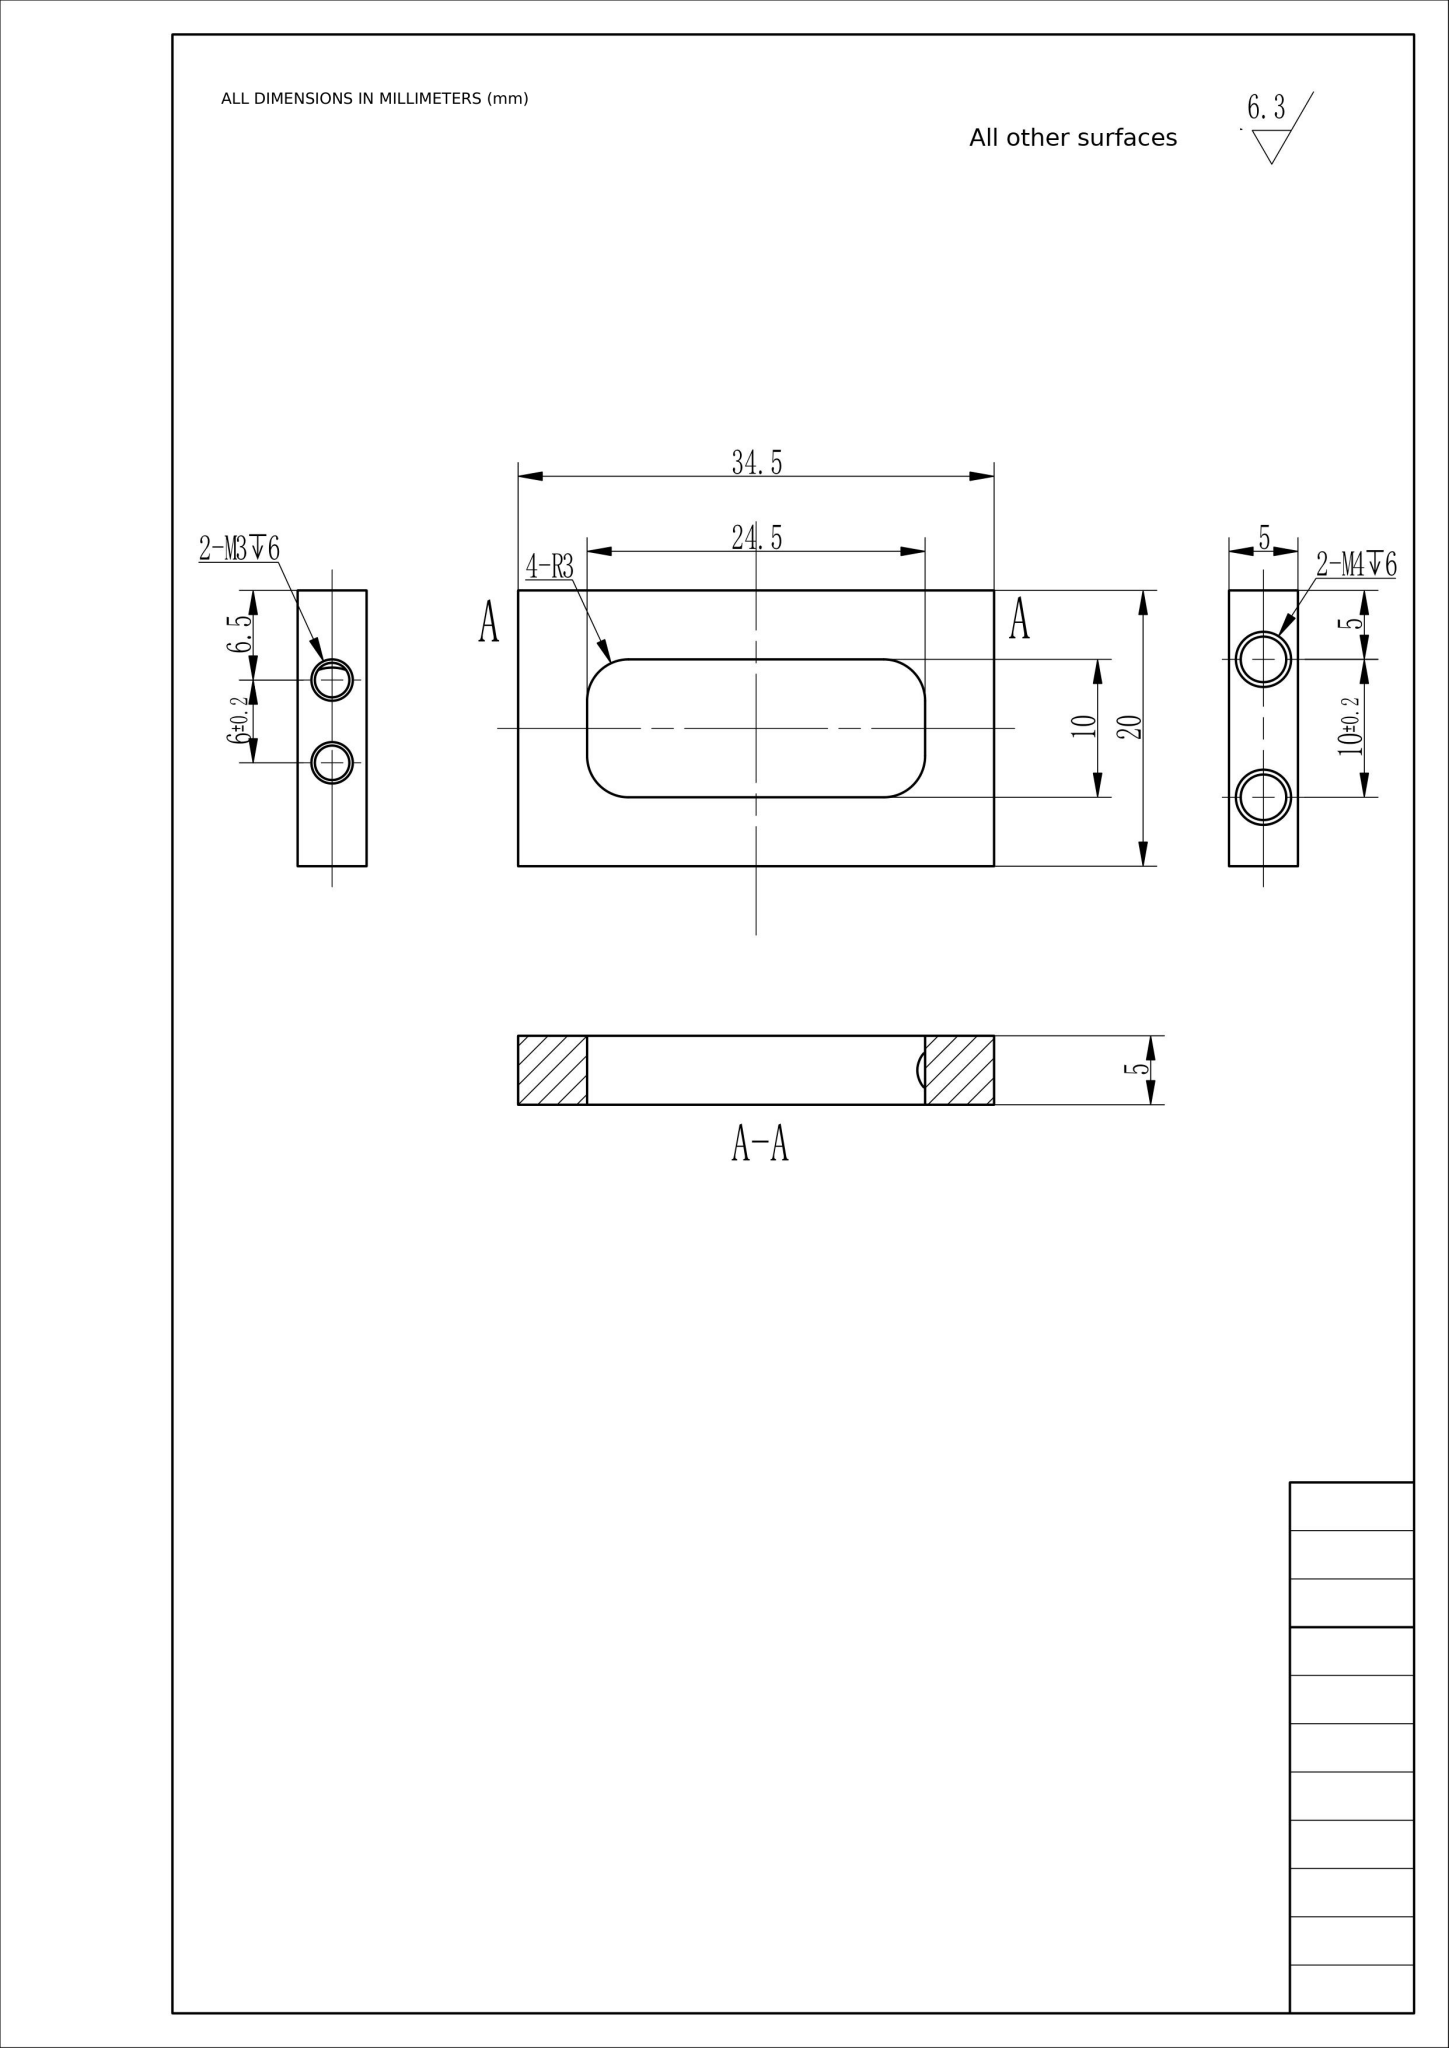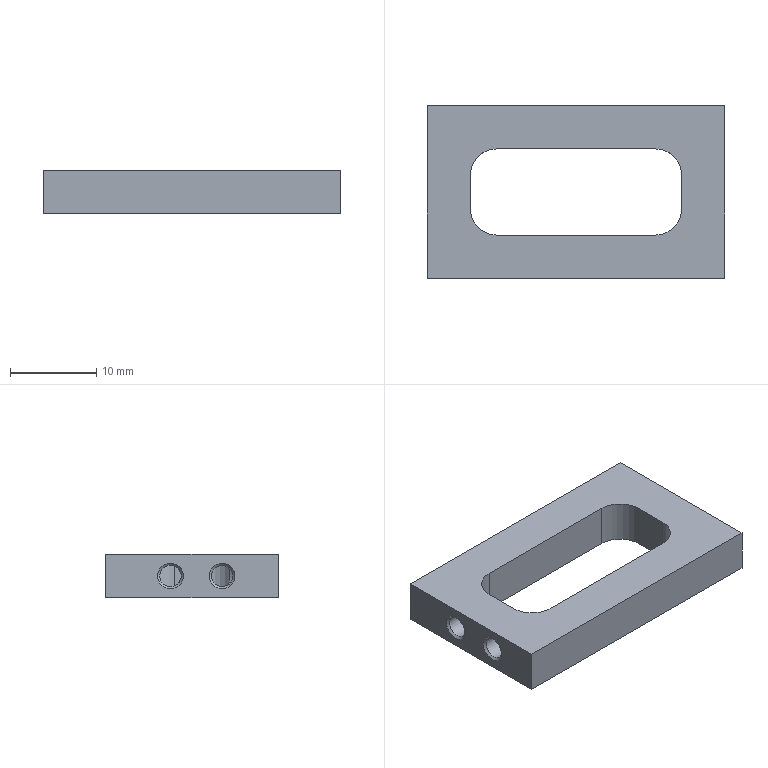Part | NX | mm | 1 solid | 25 faces | box 34.5 x 20 x 5 mm | volume 2119 mm3 | plane 10 | cylinder 8 | cone 7 | commonest cylinder face diameters 6 x4 3.3 x2 2.5 x2
STEP:
#1=CARTESIAN_POINT('',(0.,0.,0.));
#2=DIRECTION('',(0.,0.,1.));
#3=DIRECTION('',(1.,0.,0.));
#4=AXIS2_PLACEMENT_3D('',#1,#2,#3);
#5=(LENGTH_UNIT()NAMED_UNIT(*)SI_UNIT(.MILLI.,.METRE.));
#6=UNCERTAINTY_MEASURE_WITH_UNIT(LENGTH_MEASURE(0.0508),#5,'','');
#7=(NAMED_UNIT(*)PLANE_ANGLE_UNIT()SI_UNIT($,.RADIAN.));
#8=PLANE_ANGLE_MEASURE_WITH_UNIT(PLANE_ANGLE_MEASURE(0.01745),#7);
#9=DIMENSIONAL_EXPONENTS(0.,0.,0.,0.,0.,0.,0.);
#10=(CONVERSION_BASED_UNIT('',#8)NAMED_UNIT(#9)PLANE_ANGLE_UNIT());
#11=(NAMED_UNIT(*)SI_UNIT($,.STERADIAN.)SOLID_ANGLE_UNIT());
#12=(GEOMETRIC_REPRESENTATION_CONTEXT(3)GLOBAL_UNCERTAINTY_ASSIGNED_CONTEXT((#6))GLOBAL_UNIT_ASSIGNED_CONTEXT((#5,#10,#11))REPRESENTATION_CONTEXT('',''));
#13=SHAPE_REPRESENTATION('',(#4),#12);
#14=CARTESIAN_POINT('',(45.,20.,5.));
#15=VERTEX_POINT('',#14);
#16=CARTESIAN_POINT('',(45.,-0.,5.));
#17=VERTEX_POINT('',#16);
#18=CARTESIAN_POINT('',(45.,20.,5.));
#19=DIRECTION('',(0.,-1.,-0.));
#20=VECTOR('',#19,1.);
#21=LINE('',#18,#20);
#22=EDGE_CURVE('',#15,#17,#21,.T.);
#23=ORIENTED_EDGE('',*,*,#22,.T.);
#24=CARTESIAN_POINT('',(79.5,-0.,5.));
#25=VERTEX_POINT('',#24);
#26=CARTESIAN_POINT('',(79.5,-0.,5.));
#27=DIRECTION('',(-1.,0.,0.));
#28=VECTOR('',#27,1.);
#29=LINE('',#26,#28);
#30=EDGE_CURVE('',#25,#17,#29,.T.);
#31=ORIENTED_EDGE('',*,*,#30,.F.);
#32=CARTESIAN_POINT('',(79.5,20.,5.));
#33=VERTEX_POINT('',#32);
#34=CARTESIAN_POINT('',(79.5,20.,5.));
#35=DIRECTION('',(0.,-1.,-0.));
#36=VECTOR('',#35,1.);
#37=LINE('',#34,#36);
#38=EDGE_CURVE('',#33,#25,#37,.T.);
#39=ORIENTED_EDGE('',*,*,#38,.F.);
#40=CARTESIAN_POINT('',(79.5,20.,5.));
#41=DIRECTION('',(-1.,0.,0.));
#42=VECTOR('',#41,1.);
#43=LINE('',#40,#42);
#44=EDGE_CURVE('',#33,#15,#43,.T.);
#45=ORIENTED_EDGE('',*,*,#44,.T.);
#46=EDGE_LOOP('',(#23,#31,#39,#45));
#47=FACE_BOUND('',#46,.T.);
#48=CARTESIAN_POINT('',(50.,12.,5.));
#49=VERTEX_POINT('',#48);
#50=CARTESIAN_POINT('',(50.,8.,5.));
#51=VERTEX_POINT('',#50);
#52=CARTESIAN_POINT('',(50.,15.,5.));
#53=DIRECTION('',(0.,-1.,-0.));
#54=VECTOR('',#53,1.);
#55=LINE('',#52,#54);
#56=EDGE_CURVE('',#49,#51,#55,.T.);
#57=ORIENTED_EDGE('',*,*,#56,.F.);
#58=CARTESIAN_POINT('',(53.,15.,5.));
#59=VERTEX_POINT('',#58);
#60=CARTESIAN_POINT('',(53.,12.,5.));
#61=DIRECTION('',(0.,0.,-1.));
#62=DIRECTION('',(0.,1.,0.));
#63=AXIS2_PLACEMENT_3D('',#60,#61,#62);
#64=CIRCLE('',#63,3.);
#65=EDGE_CURVE('',#49,#59,#64,.T.);
#66=ORIENTED_EDGE('',*,*,#65,.T.);
#67=CARTESIAN_POINT('',(71.5,15.,5.));
#68=VERTEX_POINT('',#67);
#69=CARTESIAN_POINT('',(74.5,15.,5.));
#70=DIRECTION('',(-1.,0.,0.));
#71=VECTOR('',#70,1.);
#72=LINE('',#69,#71);
#73=EDGE_CURVE('',#68,#59,#72,.T.);
#74=ORIENTED_EDGE('',*,*,#73,.F.);
#75=CARTESIAN_POINT('',(74.5,12.,5.));
#76=VERTEX_POINT('',#75);
#77=CARTESIAN_POINT('',(71.5,12.,5.));
#78=DIRECTION('',(0.,0.,-1.));
#79=DIRECTION('',(0.,1.,0.));
#80=AXIS2_PLACEMENT_3D('',#77,#78,#79);
#81=CIRCLE('',#80,3.);
#82=EDGE_CURVE('',#68,#76,#81,.T.);
#83=ORIENTED_EDGE('',*,*,#82,.T.);
#84=CARTESIAN_POINT('',(74.5,8.,5.));
#85=VERTEX_POINT('',#84);
#86=CARTESIAN_POINT('',(74.5,5.,5.));
#87=DIRECTION('',(0.,1.,0.));
#88=VECTOR('',#87,1.);
#89=LINE('',#86,#88);
#90=EDGE_CURVE('',#85,#76,#89,.T.);
#91=ORIENTED_EDGE('',*,*,#90,.F.);
#92=CARTESIAN_POINT('',(71.5,5.,5.));
#93=VERTEX_POINT('',#92);
#94=CARTESIAN_POINT('',(71.5,8.,5.));
#95=DIRECTION('',(0.,0.,-1.));
#96=DIRECTION('',(0.,1.,0.));
#97=AXIS2_PLACEMENT_3D('',#94,#95,#96);
#98=CIRCLE('',#97,3.);
#99=EDGE_CURVE('',#85,#93,#98,.T.);
#100=ORIENTED_EDGE('',*,*,#99,.T.);
#101=CARTESIAN_POINT('',(53.,5.,5.));
#102=VERTEX_POINT('',#101);
#103=CARTESIAN_POINT('',(50.,5.,5.));
#104=DIRECTION('',(1.,0.,0.));
#105=VECTOR('',#104,1.);
#106=LINE('',#103,#105);
#107=EDGE_CURVE('',#102,#93,#106,.T.);
#108=ORIENTED_EDGE('',*,*,#107,.F.);
#109=CARTESIAN_POINT('',(53.,8.,5.));
#110=DIRECTION('',(0.,0.,-1.));
#111=DIRECTION('',(0.,1.,0.));
#112=AXIS2_PLACEMENT_3D('',#109,#110,#111);
#113=CIRCLE('',#112,3.);
#114=EDGE_CURVE('',#102,#51,#113,.T.);
#115=ORIENTED_EDGE('',*,*,#114,.T.);
#116=EDGE_LOOP('',(#57,#66,#74,#83,#91,#100,#108,#115));
#117=FACE_BOUND('',#116,.T.);
#118=CARTESIAN_POINT('',(79.5,20.,5.));
#119=DIRECTION('',(0.,0.,-1.));
#120=DIRECTION('',(0.,1.,0.));
#121=AXIS2_PLACEMENT_3D('',#118,#119,#120);
#122=PLANE('',#121);
#123=ADVANCED_FACE('',(#47,#117),#122,.F.);
#124=CARTESIAN_POINT('',(45.,0.,0.));
#125=VERTEX_POINT('',#124);
#126=CARTESIAN_POINT('',(45.,-0.,5.));
#127=DIRECTION('',(0.,0.,-1.));
#128=VECTOR('',#127,1.);
#129=LINE('',#126,#128);
#130=EDGE_CURVE('',#17,#125,#129,.T.);
#131=ORIENTED_EDGE('',*,*,#130,.T.);
#132=CARTESIAN_POINT('',(79.5,0.,0.));
#133=VERTEX_POINT('',#132);
#134=CARTESIAN_POINT('',(79.5,0.,0.));
#135=DIRECTION('',(-1.,0.,0.));
#136=VECTOR('',#135,1.);
#137=LINE('',#134,#136);
#138=EDGE_CURVE('',#133,#125,#137,.T.);
#139=ORIENTED_EDGE('',*,*,#138,.F.);
#140=CARTESIAN_POINT('',(79.5,-0.,5.));
#141=DIRECTION('',(0.,0.,-1.));
#142=VECTOR('',#141,1.);
#143=LINE('',#140,#142);
#144=EDGE_CURVE('',#25,#133,#143,.T.);
#145=ORIENTED_EDGE('',*,*,#144,.F.);
#146=ORIENTED_EDGE('',*,*,#30,.T.);
#147=EDGE_LOOP('',(#131,#139,#145,#146));
#148=FACE_OUTER_BOUND('',#147,.T.);
#149=CARTESIAN_POINT('',(79.5,-0.,5.));
#150=DIRECTION('',(0.,1.,0.));
#151=DIRECTION('',(0.,-0.,1.));
#152=AXIS2_PLACEMENT_3D('',#149,#150,#151);
#153=PLANE('',#152);
#154=ADVANCED_FACE('',(#148),#153,.F.);
#155=CARTESIAN_POINT('',(74.5,8.,0.));
#156=VERTEX_POINT('',#155);
#157=CARTESIAN_POINT('',(74.5,12.,0.));
#158=VERTEX_POINT('',#157);
#159=CARTESIAN_POINT('',(74.5,0.,0.));
#160=DIRECTION('',(0.,1.,0.));
#161=VECTOR('',#160,1.);
#162=LINE('',#159,#161);
#163=EDGE_CURVE('',#156,#158,#162,.T.);
#164=ORIENTED_EDGE('',*,*,#163,.T.);
#165=CARTESIAN_POINT('',(71.5,15.,0.));
#166=VERTEX_POINT('',#165);
#167=CARTESIAN_POINT('',(71.5,12.,0.));
#168=DIRECTION('',(0.,0.,1.));
#169=DIRECTION('',(1.,0.,0.));
#170=AXIS2_PLACEMENT_3D('',#167,#168,#169);
#171=CIRCLE('',#170,3.);
#172=EDGE_CURVE('',#158,#166,#171,.T.);
#173=ORIENTED_EDGE('',*,*,#172,.T.);
#174=CARTESIAN_POINT('',(53.,15.,0.));
#175=VERTEX_POINT('',#174);
#176=CARTESIAN_POINT('',(79.5,15.,0.));
#177=DIRECTION('',(-1.,0.,0.));
#178=VECTOR('',#177,1.);
#179=LINE('',#176,#178);
#180=EDGE_CURVE('',#166,#175,#179,.T.);
#181=ORIENTED_EDGE('',*,*,#180,.T.);
#182=CARTESIAN_POINT('',(50.,12.,0.));
#183=VERTEX_POINT('',#182);
#184=CARTESIAN_POINT('',(53.,12.,0.));
#185=DIRECTION('',(0.,0.,1.));
#186=DIRECTION('',(1.,0.,0.));
#187=AXIS2_PLACEMENT_3D('',#184,#185,#186);
#188=CIRCLE('',#187,3.);
#189=EDGE_CURVE('',#175,#183,#188,.T.);
#190=ORIENTED_EDGE('',*,*,#189,.T.);
#191=CARTESIAN_POINT('',(50.,8.,0.));
#192=VERTEX_POINT('',#191);
#193=CARTESIAN_POINT('',(50.,0.,0.));
#194=DIRECTION('',(0.,-1.,0.));
#195=VECTOR('',#194,1.);
#196=LINE('',#193,#195);
#197=EDGE_CURVE('',#183,#192,#196,.T.);
#198=ORIENTED_EDGE('',*,*,#197,.T.);
#199=CARTESIAN_POINT('',(53.,5.,0.));
#200=VERTEX_POINT('',#199);
#201=CARTESIAN_POINT('',(53.,8.,0.));
#202=DIRECTION('',(0.,0.,1.));
#203=DIRECTION('',(1.,0.,0.));
#204=AXIS2_PLACEMENT_3D('',#201,#202,#203);
#205=CIRCLE('',#204,3.);
#206=EDGE_CURVE('',#192,#200,#205,.T.);
#207=ORIENTED_EDGE('',*,*,#206,.T.);
#208=CARTESIAN_POINT('',(71.5,5.,0.));
#209=VERTEX_POINT('',#208);
#210=CARTESIAN_POINT('',(79.5,5.,0.));
#211=DIRECTION('',(1.,0.,0.));
#212=VECTOR('',#211,1.);
#213=LINE('',#210,#212);
#214=EDGE_CURVE('',#200,#209,#213,.T.);
#215=ORIENTED_EDGE('',*,*,#214,.T.);
#216=CARTESIAN_POINT('',(71.5,8.,0.));
#217=DIRECTION('',(0.,0.,1.));
#218=DIRECTION('',(1.,0.,0.));
#219=AXIS2_PLACEMENT_3D('',#216,#217,#218);
#220=CIRCLE('',#219,3.);
#221=EDGE_CURVE('',#209,#156,#220,.T.);
#222=ORIENTED_EDGE('',*,*,#221,.T.);
#223=EDGE_LOOP('',(#164,#173,#181,#190,#198,#207,#215,#222));
#224=FACE_BOUND('',#223,.T.);
#225=CARTESIAN_POINT('',(45.,20.,0.));
#226=VERTEX_POINT('',#225);
#227=CARTESIAN_POINT('',(45.,0.,0.));
#228=DIRECTION('',(0.,1.,0.));
#229=VECTOR('',#228,1.);
#230=LINE('',#227,#229);
#231=EDGE_CURVE('',#125,#226,#230,.T.);
#232=ORIENTED_EDGE('',*,*,#231,.T.);
#233=CARTESIAN_POINT('',(79.5,20.,0.));
#234=VERTEX_POINT('',#233);
#235=CARTESIAN_POINT('',(79.5,20.,0.));
#236=DIRECTION('',(-1.,0.,0.));
#237=VECTOR('',#236,1.);
#238=LINE('',#235,#237);
#239=EDGE_CURVE('',#234,#226,#238,.T.);
#240=ORIENTED_EDGE('',*,*,#239,.F.);
#241=CARTESIAN_POINT('',(79.5,0.,0.));
#242=DIRECTION('',(0.,1.,0.));
#243=VECTOR('',#242,1.);
#244=LINE('',#241,#243);
#245=EDGE_CURVE('',#133,#234,#244,.T.);
#246=ORIENTED_EDGE('',*,*,#245,.F.);
#247=ORIENTED_EDGE('',*,*,#138,.T.);
#248=EDGE_LOOP('',(#232,#240,#246,#247));
#249=FACE_BOUND('',#248,.T.);
#250=CARTESIAN_POINT('',(79.5,0.,0.));
#251=DIRECTION('',(0.,0.,1.));
#252=DIRECTION('',(1.,0.,0.));
#253=AXIS2_PLACEMENT_3D('',#250,#251,#252);
#254=PLANE('',#253);
#255=ADVANCED_FACE('',(#224,#249),#254,.F.);
#256=CARTESIAN_POINT('',(45.,20.,0.));
#257=DIRECTION('',(0.,0.,1.));
#258=VECTOR('',#257,1.);
#259=LINE('',#256,#258);
#260=EDGE_CURVE('',#226,#15,#259,.T.);
#261=ORIENTED_EDGE('',*,*,#260,.T.);
#262=ORIENTED_EDGE('',*,*,#44,.F.);
#263=CARTESIAN_POINT('',(79.5,20.,0.));
#264=DIRECTION('',(0.,0.,1.));
#265=VECTOR('',#264,1.);
#266=LINE('',#263,#265);
#267=EDGE_CURVE('',#234,#33,#266,.T.);
#268=ORIENTED_EDGE('',*,*,#267,.F.);
#269=ORIENTED_EDGE('',*,*,#239,.T.);
#270=EDGE_LOOP('',(#261,#262,#268,#269));
#271=FACE_OUTER_BOUND('',#270,.T.);
#272=CARTESIAN_POINT('',(79.5,20.,0.));
#273=DIRECTION('',(0.,-1.,0.));
#274=DIRECTION('',(0.,0.,-1.));
#275=AXIS2_PLACEMENT_3D('',#272,#273,#274);
#276=PLANE('',#275);
#277=ADVANCED_FACE('',(#271),#276,.F.);
#278=CARTESIAN_POINT('',(79.5,5.,0.5));
#279=VERTEX_POINT('',#278);
#280=CARTESIAN_POINT('',(79.5,5.,2.5));
#281=DIRECTION('',(-1.,0.,0.));
#282=DIRECTION('',(0.,0.,-1.));
#283=AXIS2_PLACEMENT_3D('',#280,#281,#282);
#284=CIRCLE('',#283,2.);
#285=EDGE_CURVE('',#279,#279,#284,.T.);
#286=ORIENTED_EDGE('',*,*,#285,.T.);
#287=EDGE_LOOP('',(#286));
#288=FACE_BOUND('',#287,.T.);
#289=CARTESIAN_POINT('',(79.5,15.,0.5));
#290=VERTEX_POINT('',#289);
#291=CARTESIAN_POINT('',(79.5,15.,2.5));
#292=DIRECTION('',(-1.,0.,0.));
#293=DIRECTION('',(0.,0.,-1.));
#294=AXIS2_PLACEMENT_3D('',#291,#292,#293);
#295=CIRCLE('',#294,2.);
#296=EDGE_CURVE('',#290,#290,#295,.T.);
#297=ORIENTED_EDGE('',*,*,#296,.T.);
#298=EDGE_LOOP('',(#297));
#299=FACE_BOUND('',#298,.T.);
#300=ORIENTED_EDGE('',*,*,#144,.T.);
#301=ORIENTED_EDGE('',*,*,#245,.T.);
#302=ORIENTED_EDGE('',*,*,#267,.T.);
#303=ORIENTED_EDGE('',*,*,#38,.T.);
#304=EDGE_LOOP('',(#300,#301,#302,#303));
#305=FACE_BOUND('',#304,.T.);
#306=CARTESIAN_POINT('',(79.5,0.,0.));
#307=DIRECTION('',(1.,0.,0.));
#308=DIRECTION('',(0.,0.,-1.));
#309=AXIS2_PLACEMENT_3D('',#306,#307,#308);
#310=PLANE('',#309);
#311=ADVANCED_FACE('',(#288,#299,#305),#310,.T.);
#312=CARTESIAN_POINT('',(45.,12.5,1.));
#313=VERTEX_POINT('',#312);
#314=CARTESIAN_POINT('',(45.,12.5,2.5));
#315=DIRECTION('',(1.,0.,0.));
#316=DIRECTION('',(0.,0.,-1.));
#317=AXIS2_PLACEMENT_3D('',#314,#315,#316);
#318=CIRCLE('',#317,1.5);
#319=EDGE_CURVE('',#313,#313,#318,.T.);
#320=ORIENTED_EDGE('',*,*,#319,.T.);
#321=EDGE_LOOP('',(#320));
#322=FACE_BOUND('',#321,.T.);
#323=CARTESIAN_POINT('',(45.,6.5,1.));
#324=VERTEX_POINT('',#323);
#325=CARTESIAN_POINT('',(45.,6.5,2.5));
#326=DIRECTION('',(1.,0.,0.));
#327=DIRECTION('',(0.,0.,-1.));
#328=AXIS2_PLACEMENT_3D('',#325,#326,#327);
#329=CIRCLE('',#328,1.5);
#330=EDGE_CURVE('',#324,#324,#329,.T.);
#331=ORIENTED_EDGE('',*,*,#330,.T.);
#332=EDGE_LOOP('',(#331));
#333=FACE_BOUND('',#332,.T.);
#334=ORIENTED_EDGE('',*,*,#130,.F.);
#335=ORIENTED_EDGE('',*,*,#22,.F.);
#336=ORIENTED_EDGE('',*,*,#260,.F.);
#337=ORIENTED_EDGE('',*,*,#231,.F.);
#338=EDGE_LOOP('',(#334,#335,#336,#337));
#339=FACE_BOUND('',#338,.T.);
#340=CARTESIAN_POINT('',(45.,0.,0.));
#341=DIRECTION('',(1.,0.,0.));
#342=DIRECTION('',(0.,0.,-1.));
#343=AXIS2_PLACEMENT_3D('',#340,#341,#342);
#344=PLANE('',#343);
#345=ADVANCED_FACE('',(#322,#333,#339),#344,.F.);
#346=CARTESIAN_POINT('',(50.,12.,1.354));
#347=VERTEX_POINT('',#346);
#348=CARTESIAN_POINT('',(50.,12.,5.));
#349=DIRECTION('',(0.,-0.,1.));
#350=VECTOR('',#349,1.);
#351=LINE('',#348,#350);
#352=EDGE_CURVE('',#183,#347,#351,.T.);
#353=ORIENTED_EDGE('',*,*,#352,.T.);
#354=CARTESIAN_POINT('',(50.,12.,3.646));
#355=VERTEX_POINT('',#354);
#356=CARTESIAN_POINT('',(50.,12.5,2.5));
#357=DIRECTION('',(-1.,0.,0.));
#358=DIRECTION('',(0.,0.,1.));
#359=AXIS2_PLACEMENT_3D('',#356,#357,#358);
#360=CIRCLE('',#359,1.25);
#361=EDGE_CURVE('',#347,#355,#360,.T.);
#362=ORIENTED_EDGE('',*,*,#361,.T.);
#363=CARTESIAN_POINT('',(50.,12.,5.));
#364=DIRECTION('',(0.,-0.,1.));
#365=VECTOR('',#364,1.);
#366=LINE('',#363,#365);
#367=EDGE_CURVE('',#355,#49,#366,.T.);
#368=ORIENTED_EDGE('',*,*,#367,.T.);
#369=ORIENTED_EDGE('',*,*,#56,.T.);
#370=CARTESIAN_POINT('',(50.,8.,-0.));
#371=DIRECTION('',(0.,0.,-1.));
#372=VECTOR('',#371,1.);
#373=LINE('',#370,#372);
#374=EDGE_CURVE('',#51,#192,#373,.T.);
#375=ORIENTED_EDGE('',*,*,#374,.T.);
#376=ORIENTED_EDGE('',*,*,#197,.F.);
#377=EDGE_LOOP('',(#353,#362,#368,#369,#375,#376));
#378=FACE_OUTER_BOUND('',#377,.T.);
#379=CARTESIAN_POINT('',(50.,15.,-74.5));
#380=DIRECTION('',(-1.,0.,0.));
#381=DIRECTION('',(0.,0.,1.));
#382=AXIS2_PLACEMENT_3D('',#379,#380,#381);
#383=PLANE('',#382);
#384=ADVANCED_FACE('',(#378),#383,.F.);
#385=ORIENTED_EDGE('',*,*,#107,.T.);
#386=CARTESIAN_POINT('',(71.5,5.,-0.));
#387=DIRECTION('',(0.,0.,-1.));
#388=VECTOR('',#387,1.);
#389=LINE('',#386,#388);
#390=EDGE_CURVE('',#93,#209,#389,.T.);
#391=ORIENTED_EDGE('',*,*,#390,.T.);
#392=ORIENTED_EDGE('',*,*,#214,.F.);
#393=CARTESIAN_POINT('',(53.,5.,5.));
#394=DIRECTION('',(0.,-0.,1.));
#395=VECTOR('',#394,1.);
#396=LINE('',#393,#395);
#397=EDGE_CURVE('',#200,#102,#396,.T.);
#398=ORIENTED_EDGE('',*,*,#397,.T.);
#399=EDGE_LOOP('',(#385,#391,#392,#398));
#400=FACE_OUTER_BOUND('',#399,.T.);
#401=CARTESIAN_POINT('',(50.,5.,-74.5));
#402=DIRECTION('',(0.,-1.,-0.));
#403=DIRECTION('',(0.,0.,-1.));
#404=AXIS2_PLACEMENT_3D('',#401,#402,#403);
#405=PLANE('',#404);
#406=ADVANCED_FACE('',(#400),#405,.F.);
#407=ORIENTED_EDGE('',*,*,#163,.F.);
#408=CARTESIAN_POINT('',(74.5,8.,5.));
#409=DIRECTION('',(0.,-0.,1.));
#410=VECTOR('',#409,1.);
#411=LINE('',#408,#410);
#412=EDGE_CURVE('',#156,#85,#411,.T.);
#413=ORIENTED_EDGE('',*,*,#412,.T.);
#414=ORIENTED_EDGE('',*,*,#90,.T.);
#415=CARTESIAN_POINT('',(74.5,12.,-0.));
#416=DIRECTION('',(0.,0.,-1.));
#417=VECTOR('',#416,1.);
#418=LINE('',#415,#417);
#419=EDGE_CURVE('',#76,#158,#418,.T.);
#420=ORIENTED_EDGE('',*,*,#419,.T.);
#421=EDGE_LOOP('',(#407,#413,#414,#420));
#422=FACE_OUTER_BOUND('',#421,.T.);
#423=CARTESIAN_POINT('',(74.5,5.,-74.5));
#424=DIRECTION('',(1.,0.,0.));
#425=DIRECTION('',(0.,0.,-1.));
#426=AXIS2_PLACEMENT_3D('',#423,#424,#425);
#427=PLANE('',#426);
#428=ADVANCED_FACE('',(#422),#427,.F.);
#429=ORIENTED_EDGE('',*,*,#180,.F.);
#430=CARTESIAN_POINT('',(71.5,15.,5.));
#431=DIRECTION('',(0.,-0.,1.));
#432=VECTOR('',#431,1.);
#433=LINE('',#430,#432);
#434=EDGE_CURVE('',#166,#68,#433,.T.);
#435=ORIENTED_EDGE('',*,*,#434,.T.);
#436=ORIENTED_EDGE('',*,*,#73,.T.);
#437=CARTESIAN_POINT('',(53.,15.,0.));
#438=DIRECTION('',(0.,0.,-1.));
#439=VECTOR('',#438,1.);
#440=LINE('',#437,#439);
#441=EDGE_CURVE('',#59,#175,#440,.T.);
#442=ORIENTED_EDGE('',*,*,#441,.T.);
#443=EDGE_LOOP('',(#429,#435,#436,#442));
#444=FACE_OUTER_BOUND('',#443,.T.);
#445=CARTESIAN_POINT('',(74.5,15.,-74.5));
#446=DIRECTION('',(0.,1.,0.));
#447=DIRECTION('',(0.,-0.,1.));
#448=AXIS2_PLACEMENT_3D('',#445,#446,#447);
#449=PLANE('',#448);
#450=ADVANCED_FACE('',(#444),#449,.F.);
#451=ORIENTED_EDGE('',*,*,#99,.F.);
#452=ORIENTED_EDGE('',*,*,#412,.F.);
#453=ORIENTED_EDGE('',*,*,#221,.F.);
#454=ORIENTED_EDGE('',*,*,#390,.F.);
#455=EDGE_LOOP('',(#451,#452,#453,#454));
#456=FACE_OUTER_BOUND('',#455,.T.);
#457=CARTESIAN_POINT('',(71.5,8.,-74.5));
#458=DIRECTION('',(0.,-0.,1.));
#459=DIRECTION('',(0.,-1.,0.));
#460=AXIS2_PLACEMENT_3D('',#457,#458,#459);
#461=CYLINDRICAL_SURFACE('',#460,3.);
#462=ADVANCED_FACE('',(#456),#461,.F.);
#463=ORIENTED_EDGE('',*,*,#82,.F.);
#464=ORIENTED_EDGE('',*,*,#434,.F.);
#465=ORIENTED_EDGE('',*,*,#172,.F.);
#466=ORIENTED_EDGE('',*,*,#419,.F.);
#467=EDGE_LOOP('',(#463,#464,#465,#466));
#468=FACE_OUTER_BOUND('',#467,.T.);
#469=CARTESIAN_POINT('',(71.5,12.,-74.5));
#470=DIRECTION('',(0.,-0.,1.));
#471=DIRECTION('',(0.,-1.,0.));
#472=AXIS2_PLACEMENT_3D('',#469,#470,#471);
#473=CYLINDRICAL_SURFACE('',#472,3.);
#474=ADVANCED_FACE('',(#468),#473,.F.);
#475=ORIENTED_EDGE('',*,*,#367,.F.);
#476=CARTESIAN_POINT('',(50.,12.,3.646));
#477=CARTESIAN_POINT('',(50.,12.12,3.698));
#478=CARTESIAN_POINT('',(50.008,12.251,3.732));
#479=CARTESIAN_POINT('',(50.024,12.381,3.744));
#480=CARTESIAN_POINT('',(50.041,12.51,3.757));
#481=CARTESIAN_POINT('',(50.067,12.642,3.748));
#482=CARTESIAN_POINT('',(50.1,12.767,3.721));
#483=CARTESIAN_POINT('',(50.133,12.893,3.694));
#484=CARTESIAN_POINT('',(50.174,13.015,3.646));
#485=CARTESIAN_POINT('',(50.219,13.125,3.583));
#486=CARTESIAN_POINT('',(50.267,13.245,3.513));
#487=CARTESIAN_POINT('',(50.321,13.353,3.424));
#488=CARTESIAN_POINT('',(50.37,13.444,3.319));
#489=CARTESIAN_POINT('',(50.424,13.542,3.207));
#490=CARTESIAN_POINT('',(50.475,13.621,3.074));
#491=CARTESIAN_POINT('',(50.511,13.674,2.929));
#492=CARTESIAN_POINT('',(50.537,13.714,2.82));
#493=CARTESIAN_POINT('',(50.556,13.739,2.701));
#494=CARTESIAN_POINT('',(50.561,13.747,2.582));
#495=CARTESIAN_POINT('',(50.567,13.755,2.463));
#496=CARTESIAN_POINT('',(50.56,13.745,2.34));
#497=CARTESIAN_POINT('',(50.542,13.719,2.225));
#498=CARTESIAN_POINT('',(50.524,13.694,2.114));
#499=CARTESIAN_POINT('',(50.496,13.654,2.007));
#500=CARTESIAN_POINT('',(50.463,13.602,1.91));
#501=CARTESIAN_POINT('',(50.426,13.543,1.8));
#502=CARTESIAN_POINT('',(50.382,13.468,1.7));
#503=CARTESIAN_POINT('',(50.337,13.381,1.613));
#504=CARTESIAN_POINT('',(50.284,13.28,1.513));
#505=CARTESIAN_POINT('',(50.23,13.16,1.429));
#506=CARTESIAN_POINT('',(50.182,13.03,1.368));
#507=CARTESIAN_POINT('',(50.133,12.895,1.305));
#508=CARTESIAN_POINT('',(50.089,12.743,1.264));
#509=CARTESIAN_POINT('',(50.059,12.59,1.253));
#510=CARTESIAN_POINT('',(50.031,12.45,1.243));
#511=CARTESIAN_POINT('',(50.012,12.305,1.257));
#512=CARTESIAN_POINT('',(50.005,12.168,1.295));
#513=CARTESIAN_POINT('',(50.002,12.111,1.311));
#514=CARTESIAN_POINT('',(50.,12.054,1.331));
#515=CARTESIAN_POINT('',(50.,12.,1.354));
#516=B_SPLINE_CURVE_WITH_KNOTS('',3,(#476,#477,#478,#479,#480,#481,#482,#483,#484,#485,#486,#487,#488,#489,#490,#491,#492,#493,#494,#495,#496,#497,#498,#499,#500,#501,#502,#503,#504,#505,#506,#507,#508,#509,#510,#511,#512,#513,#514,#515),.UNSPECIFIED.,.F.,.F.,(4,3,3,3,3,3,3,3,3,3,3,3,3,4),(0.,0.07747,0.1549,0.2338,0.3204,0.414,0.4842,0.5547,0.6224,0.6989,0.7884,0.8813,0.9654,1.),.UNSPECIFIED.);
#517=EDGE_CURVE('',#355,#347,#516,.T.);
#518=ORIENTED_EDGE('',*,*,#517,.T.);
#519=ORIENTED_EDGE('',*,*,#352,.F.);
#520=ORIENTED_EDGE('',*,*,#189,.F.);
#521=ORIENTED_EDGE('',*,*,#441,.F.);
#522=ORIENTED_EDGE('',*,*,#65,.F.);
#523=EDGE_LOOP('',(#475,#518,#519,#520,#521,#522));
#524=FACE_OUTER_BOUND('',#523,.T.);
#525=CARTESIAN_POINT('',(53.,12.,-74.5));
#526=DIRECTION('',(0.,-0.,1.));
#527=DIRECTION('',(0.,-1.,0.));
#528=AXIS2_PLACEMENT_3D('',#525,#526,#527);
#529=CYLINDRICAL_SURFACE('',#528,3.);
#530=ADVANCED_FACE('',(#524),#529,.F.);
#531=CARTESIAN_POINT('',(51.,5.764,3.51));
#532=VERTEX_POINT('',#531);
#533=CARTESIAN_POINT('',(51.,5.764,1.49));
#534=VERTEX_POINT('',#533);
#535=CARTESIAN_POINT('',(51.,5.764,3.51));
#536=CARTESIAN_POINT('',(50.859,5.89,3.602));
#537=CARTESIAN_POINT('',(50.72,6.04,3.675));
#538=CARTESIAN_POINT('',(50.596,6.205,3.715));
#539=CARTESIAN_POINT('',(50.499,6.335,3.746));
#540=CARTESIAN_POINT('',(50.41,6.478,3.758));
#541=CARTESIAN_POINT('',(50.334,6.624,3.744));
#542=CARTESIAN_POINT('',(50.259,6.77,3.729));
#543=CARTESIAN_POINT('',(50.195,6.925,3.686));
#544=CARTESIAN_POINT('',(50.149,7.067,3.614));
#545=CARTESIAN_POINT('',(50.109,7.189,3.552));
#546=CARTESIAN_POINT('',(50.08,7.305,3.466));
#547=CARTESIAN_POINT('',(50.06,7.403,3.364));
#548=CARTESIAN_POINT('',(50.041,7.495,3.268));
#549=CARTESIAN_POINT('',(50.03,7.573,3.155));
#550=CARTESIAN_POINT('',(50.023,7.63,3.034));
#551=CARTESIAN_POINT('',(50.016,7.688,2.911));
#552=CARTESIAN_POINT('',(50.012,7.727,2.777));
#553=CARTESIAN_POINT('',(50.011,7.742,2.641));
#554=CARTESIAN_POINT('',(50.01,7.758,2.504));
#555=CARTESIAN_POINT('',(50.01,7.75,2.361));
#556=CARTESIAN_POINT('',(50.013,7.72,2.226));
#557=CARTESIAN_POINT('',(50.016,7.689,2.09));
#558=CARTESIAN_POINT('',(50.021,7.635,1.957));
#559=CARTESIAN_POINT('',(50.032,7.561,1.839));
#560=CARTESIAN_POINT('',(50.043,7.488,1.722));
#561=CARTESIAN_POINT('',(50.06,7.394,1.616));
#562=CARTESIAN_POINT('',(50.085,7.289,1.53));
#563=CARTESIAN_POINT('',(50.111,7.186,1.447));
#564=CARTESIAN_POINT('',(50.145,7.069,1.38));
#565=CARTESIAN_POINT('',(50.19,6.95,1.334));
#566=CARTESIAN_POINT('',(50.234,6.832,1.288));
#567=CARTESIAN_POINT('',(50.289,6.708,1.262));
#568=CARTESIAN_POINT('',(50.352,6.589,1.253));
#569=CARTESIAN_POINT('',(50.42,6.462,1.244));
#570=CARTESIAN_POINT('',(50.499,6.337,1.255));
#571=CARTESIAN_POINT('',(50.584,6.222,1.281));
#572=CARTESIAN_POINT('',(50.711,6.05,1.321));
#573=CARTESIAN_POINT('',(50.854,5.894,1.395));
#574=CARTESIAN_POINT('',(51.,5.764,1.49));
#575=B_SPLINE_CURVE_WITH_KNOTS('',3,(#535,#536,#537,#538,#539,#540,#541,#542,#543,#544,#545,#546,#547,#548,#549,#550,#551,#552,#553,#554,#555,#556,#557,#558,#559,#560,#561,#562,#563,#564,#565,#566,#567,#568,#569,#570,#571,#572,#573,#574),.UNSPECIFIED.,.F.,.F.,(4,3,3,3,3,3,3,3,3,3,3,3,3,4),(0.,0.1055,0.1877,0.2709,0.3422,0.409,0.4769,0.5461,0.6156,0.6846,0.752,0.819,0.8911,1.),.UNSPECIFIED.);
#576=EDGE_CURVE('',#532,#534,#575,.T.);
#577=ORIENTED_EDGE('',*,*,#576,.T.);
#578=CARTESIAN_POINT('',(51.,5.764,1.49));
#579=CARTESIAN_POINT('',(51.088,5.685,1.73));
#580=CARTESIAN_POINT('',(51.164,5.627,1.987));
#581=CARTESIAN_POINT('',(51.193,5.605,2.252));
#582=CARTESIAN_POINT('',(51.217,5.587,2.469));
#583=CARTESIAN_POINT('',(51.208,5.594,2.694));
#584=CARTESIAN_POINT('',(51.17,5.623,2.907));
#585=CARTESIAN_POINT('',(51.133,5.651,3.116));
#586=CARTESIAN_POINT('',(51.071,5.701,3.318));
#587=CARTESIAN_POINT('',(51.,5.764,3.51));
#588=B_SPLINE_CURVE_WITH_KNOTS('',3,(#578,#579,#580,#581,#582,#583,#584,#585,#586,#587),.UNSPECIFIED.,.F.,.F.,(4,3,3,4),(0.,0.3838,0.6952,1.),.UNSPECIFIED.);
#589=EDGE_CURVE('',#534,#532,#588,.T.);
#590=ORIENTED_EDGE('',*,*,#589,.T.);
#591=EDGE_LOOP('',(#577,#590));
#592=FACE_BOUND('',#591,.T.);
#593=ORIENTED_EDGE('',*,*,#114,.F.);
#594=ORIENTED_EDGE('',*,*,#397,.F.);
#595=ORIENTED_EDGE('',*,*,#206,.F.);
#596=ORIENTED_EDGE('',*,*,#374,.F.);
#597=EDGE_LOOP('',(#593,#594,#595,#596));
#598=FACE_BOUND('',#597,.T.);
#599=CARTESIAN_POINT('',(53.,8.,-74.5));
#600=DIRECTION('',(0.,-0.,1.));
#601=DIRECTION('',(0.,-1.,0.));
#602=AXIS2_PLACEMENT_3D('',#599,#600,#601);
#603=CYLINDRICAL_SURFACE('',#602,3.);
#604=ADVANCED_FACE('',(#592,#598),#603,.F.);
#605=CARTESIAN_POINT('',(74.5,15.,4.15));
#606=VERTEX_POINT('',#605);
#607=CARTESIAN_POINT('',(74.5,15.,2.5));
#608=DIRECTION('',(1.,0.,0.));
#609=DIRECTION('',(0.,0.,1.));
#610=AXIS2_PLACEMENT_3D('',#607,#608,#609);
#611=CIRCLE('',#610,1.65);
#612=EDGE_CURVE('',#606,#606,#611,.T.);
#613=ORIENTED_EDGE('',*,*,#612,.T.);
#614=EDGE_LOOP('',(#613));
#615=FACE_BOUND('',#614,.T.);
#616=CARTESIAN_POINT('',(73.509,15.,2.5));
#617=VERTEX_POINT('',#616);
#618=VERTEX_LOOP('',#617);
#619=FACE_BOUND('',#618,.T.);
#620=CARTESIAN_POINT('',(74.5,15.,2.5));
#621=DIRECTION('',(1.,0.,0.));
#622=DIRECTION('',(0.,0.,-1.));
#623=AXIS2_PLACEMENT_3D('',#620,#621,#622);
#624=CONICAL_SURFACE('',#623,1.65,59.);
#625=ADVANCED_FACE('',(#615,#619),#624,.F.);
#626=CARTESIAN_POINT('',(79.15,15.,0.85));
#627=VERTEX_POINT('',#626);
#628=CARTESIAN_POINT('',(79.15,15.,2.5));
#629=DIRECTION('',(1.,0.,0.));
#630=DIRECTION('',(0.,0.,-1.));
#631=AXIS2_PLACEMENT_3D('',#628,#629,#630);
#632=CIRCLE('',#631,1.65);
#633=EDGE_CURVE('',#627,#627,#632,.T.);
#634=ORIENTED_EDGE('',*,*,#633,.T.);
#635=EDGE_LOOP('',(#634));
#636=FACE_BOUND('',#635,.T.);
#637=ORIENTED_EDGE('',*,*,#612,.F.);
#638=EDGE_LOOP('',(#637));
#639=FACE_BOUND('',#638,.T.);
#640=CARTESIAN_POINT('',(79.5,15.,2.5));
#641=DIRECTION('',(-1.,0.,0.));
#642=DIRECTION('',(0.,0.,1.));
#643=AXIS2_PLACEMENT_3D('',#640,#641,#642);
#644=CYLINDRICAL_SURFACE('',#643,1.65);
#645=ADVANCED_FACE('',(#636,#639),#644,.F.);
#646=ORIENTED_EDGE('',*,*,#633,.F.);
#647=EDGE_LOOP('',(#646));
#648=FACE_BOUND('',#647,.T.);
#649=ORIENTED_EDGE('',*,*,#296,.F.);
#650=EDGE_LOOP('',(#649));
#651=FACE_BOUND('',#650,.T.);
#652=CARTESIAN_POINT('',(79.5,15.,2.5));
#653=DIRECTION('',(1.,0.,0.));
#654=DIRECTION('',(-0.,0.,-1.));
#655=AXIS2_PLACEMENT_3D('',#652,#653,#654);
#656=CONICAL_SURFACE('',#655,2.,45.);
#657=ADVANCED_FACE('',(#648,#651),#656,.F.);
#658=CARTESIAN_POINT('',(74.5,5.,4.15));
#659=VERTEX_POINT('',#658);
#660=CARTESIAN_POINT('',(74.5,5.,2.5));
#661=DIRECTION('',(1.,0.,0.));
#662=DIRECTION('',(0.,0.,1.));
#663=AXIS2_PLACEMENT_3D('',#660,#661,#662);
#664=CIRCLE('',#663,1.65);
#665=EDGE_CURVE('',#659,#659,#664,.T.);
#666=ORIENTED_EDGE('',*,*,#665,.T.);
#667=EDGE_LOOP('',(#666));
#668=FACE_BOUND('',#667,.T.);
#669=CARTESIAN_POINT('',(73.509,5.,2.5));
#670=VERTEX_POINT('',#669);
#671=VERTEX_LOOP('',#670);
#672=FACE_BOUND('',#671,.T.);
#673=CARTESIAN_POINT('',(74.5,5.,2.5));
#674=DIRECTION('',(1.,0.,0.));
#675=DIRECTION('',(0.,0.,-1.));
#676=AXIS2_PLACEMENT_3D('',#673,#674,#675);
#677=CONICAL_SURFACE('',#676,1.65,59.);
#678=ADVANCED_FACE('',(#668,#672),#677,.F.);
#679=CARTESIAN_POINT('',(79.15,5.,0.85));
#680=VERTEX_POINT('',#679);
#681=CARTESIAN_POINT('',(79.15,5.,2.5));
#682=DIRECTION('',(1.,0.,0.));
#683=DIRECTION('',(0.,0.,-1.));
#684=AXIS2_PLACEMENT_3D('',#681,#682,#683);
#685=CIRCLE('',#684,1.65);
#686=EDGE_CURVE('',#680,#680,#685,.T.);
#687=ORIENTED_EDGE('',*,*,#686,.T.);
#688=EDGE_LOOP('',(#687));
#689=FACE_BOUND('',#688,.T.);
#690=ORIENTED_EDGE('',*,*,#665,.F.);
#691=EDGE_LOOP('',(#690));
#692=FACE_BOUND('',#691,.T.);
#693=CARTESIAN_POINT('',(79.5,5.,2.5));
#694=DIRECTION('',(-1.,0.,0.));
#695=DIRECTION('',(0.,0.,1.));
#696=AXIS2_PLACEMENT_3D('',#693,#694,#695);
#697=CYLINDRICAL_SURFACE('',#696,1.65);
#698=ADVANCED_FACE('',(#689,#692),#697,.F.);
#699=ORIENTED_EDGE('',*,*,#686,.F.);
#700=EDGE_LOOP('',(#699));
#701=FACE_BOUND('',#700,.T.);
#702=ORIENTED_EDGE('',*,*,#285,.F.);
#703=EDGE_LOOP('',(#702));
#704=FACE_BOUND('',#703,.T.);
#705=CARTESIAN_POINT('',(79.5,5.,2.5));
#706=DIRECTION('',(1.,0.,0.));
#707=DIRECTION('',(-0.,0.,-1.));
#708=AXIS2_PLACEMENT_3D('',#705,#706,#707);
#709=CONICAL_SURFACE('',#708,2.,45.);
#710=ADVANCED_FACE('',(#701,#704),#709,.F.);
#711=CARTESIAN_POINT('',(51.,6.5,2.5));
#712=DIRECTION('',(-1.,0.,0.));
#713=DIRECTION('',(0.,0.,-1.));
#714=AXIS2_PLACEMENT_3D('',#711,#712,#713);
#715=CIRCLE('',#714,1.25);
#716=EDGE_CURVE('',#534,#532,#715,.T.);
#717=ORIENTED_EDGE('',*,*,#716,.T.);
#718=ORIENTED_EDGE('',*,*,#589,.F.);
#719=EDGE_LOOP('',(#717,#718));
#720=FACE_OUTER_BOUND('',#719,.T.);
#721=CARTESIAN_POINT('',(51.,6.5,2.5));
#722=DIRECTION('',(-1.,0.,0.));
#723=DIRECTION('',(0.,0.,1.));
#724=AXIS2_PLACEMENT_3D('',#721,#722,#723);
#725=CONICAL_SURFACE('',#724,1.25,59.);
#726=ADVANCED_FACE('',(#720),#725,.F.);
#727=CARTESIAN_POINT('',(45.25,6.5,1.25));
#728=VERTEX_POINT('',#727);
#729=CARTESIAN_POINT('',(45.25,6.5,2.5));
#730=DIRECTION('',(-1.,0.,0.));
#731=DIRECTION('',(0.,0.,-1.));
#732=AXIS2_PLACEMENT_3D('',#729,#730,#731);
#733=CIRCLE('',#732,1.25);
#734=EDGE_CURVE('',#728,#728,#733,.T.);
#735=ORIENTED_EDGE('',*,*,#734,.T.);
#736=EDGE_LOOP('',(#735));
#737=FACE_BOUND('',#736,.T.);
#738=ORIENTED_EDGE('',*,*,#716,.F.);
#739=ORIENTED_EDGE('',*,*,#576,.F.);
#740=EDGE_LOOP('',(#738,#739));
#741=FACE_BOUND('',#740,.T.);
#742=CARTESIAN_POINT('',(45.,6.5,2.5));
#743=DIRECTION('',(1.,0.,0.));
#744=DIRECTION('',(0.,0.,-1.));
#745=AXIS2_PLACEMENT_3D('',#742,#743,#744);
#746=CYLINDRICAL_SURFACE('',#745,1.25);
#747=ADVANCED_FACE('',(#737,#741),#746,.F.);
#748=ORIENTED_EDGE('',*,*,#734,.F.);
#749=EDGE_LOOP('',(#748));
#750=FACE_BOUND('',#749,.T.);
#751=ORIENTED_EDGE('',*,*,#330,.F.);
#752=EDGE_LOOP('',(#751));
#753=FACE_BOUND('',#752,.T.);
#754=CARTESIAN_POINT('',(45.,6.5,2.5));
#755=DIRECTION('',(-1.,0.,0.));
#756=DIRECTION('',(0.,0.,1.));
#757=AXIS2_PLACEMENT_3D('',#754,#755,#756);
#758=CONICAL_SURFACE('',#757,1.5,45.);
#759=ADVANCED_FACE('',(#750,#753),#758,.F.);
#760=CARTESIAN_POINT('',(45.25,12.5,1.25));
#761=VERTEX_POINT('',#760);
#762=CARTESIAN_POINT('',(45.25,12.5,2.5));
#763=DIRECTION('',(-1.,0.,0.));
#764=DIRECTION('',(0.,0.,-1.));
#765=AXIS2_PLACEMENT_3D('',#762,#763,#764);
#766=CIRCLE('',#765,1.25);
#767=EDGE_CURVE('',#761,#761,#766,.T.);
#768=ORIENTED_EDGE('',*,*,#767,.T.);
#769=EDGE_LOOP('',(#768));
#770=FACE_BOUND('',#769,.T.);
#771=ORIENTED_EDGE('',*,*,#517,.F.);
#772=ORIENTED_EDGE('',*,*,#361,.F.);
#773=EDGE_LOOP('',(#771,#772));
#774=FACE_BOUND('',#773,.T.);
#775=CARTESIAN_POINT('',(45.,12.5,2.5));
#776=DIRECTION('',(1.,0.,0.));
#777=DIRECTION('',(0.,0.,-1.));
#778=AXIS2_PLACEMENT_3D('',#775,#776,#777);
#779=CYLINDRICAL_SURFACE('',#778,1.25);
#780=ADVANCED_FACE('',(#770,#774),#779,.F.);
#781=ORIENTED_EDGE('',*,*,#767,.F.);
#782=EDGE_LOOP('',(#781));
#783=FACE_BOUND('',#782,.T.);
#784=ORIENTED_EDGE('',*,*,#319,.F.);
#785=EDGE_LOOP('',(#784));
#786=FACE_BOUND('',#785,.T.);
#787=CARTESIAN_POINT('',(45.,12.5,2.5));
#788=DIRECTION('',(-1.,0.,0.));
#789=DIRECTION('',(0.,0.,1.));
#790=AXIS2_PLACEMENT_3D('',#787,#788,#789);
#791=CONICAL_SURFACE('',#790,1.5,45.);
#792=ADVANCED_FACE('',(#783,#786),#791,.F.);
#793=CLOSED_SHELL('',(#123,#154,#255,#277,#311,#345,#384,#406,#428,#450,#462,#474,#530,#604,#625,#645,#657,#678,#698,#710,#726,#747,#759,#780,#792));
#794=MANIFOLD_SOLID_BREP('',#793);
#795=ADVANCED_BREP_SHAPE_REPRESENTATION('',(#794),#12);
#796=SHAPE_REPRESENTATION_RELATIONSHIP('','',#13,#795);
#797=PRESENTATION_LAYER_ASSIGNMENT('','',(#794));
#798=COLOUR_RGB('',1.,0.6,0.);
#799=FILL_AREA_STYLE_COLOUR('',#798);
#800=FILL_AREA_STYLE('',(#799));
#801=SURFACE_STYLE_FILL_AREA(#800);
#802=SURFACE_SIDE_STYLE('',(#801));
#803=SURFACE_STYLE_USAGE(.BOTH.,#802);
#804=PRESENTATION_STYLE_ASSIGNMENT((#803));
#805=STYLED_ITEM('',(#804),#794);
#806=MECHANICAL_DESIGN_GEOMETRIC_PRESENTATION_REPRESENTATION('',(#805),#12);